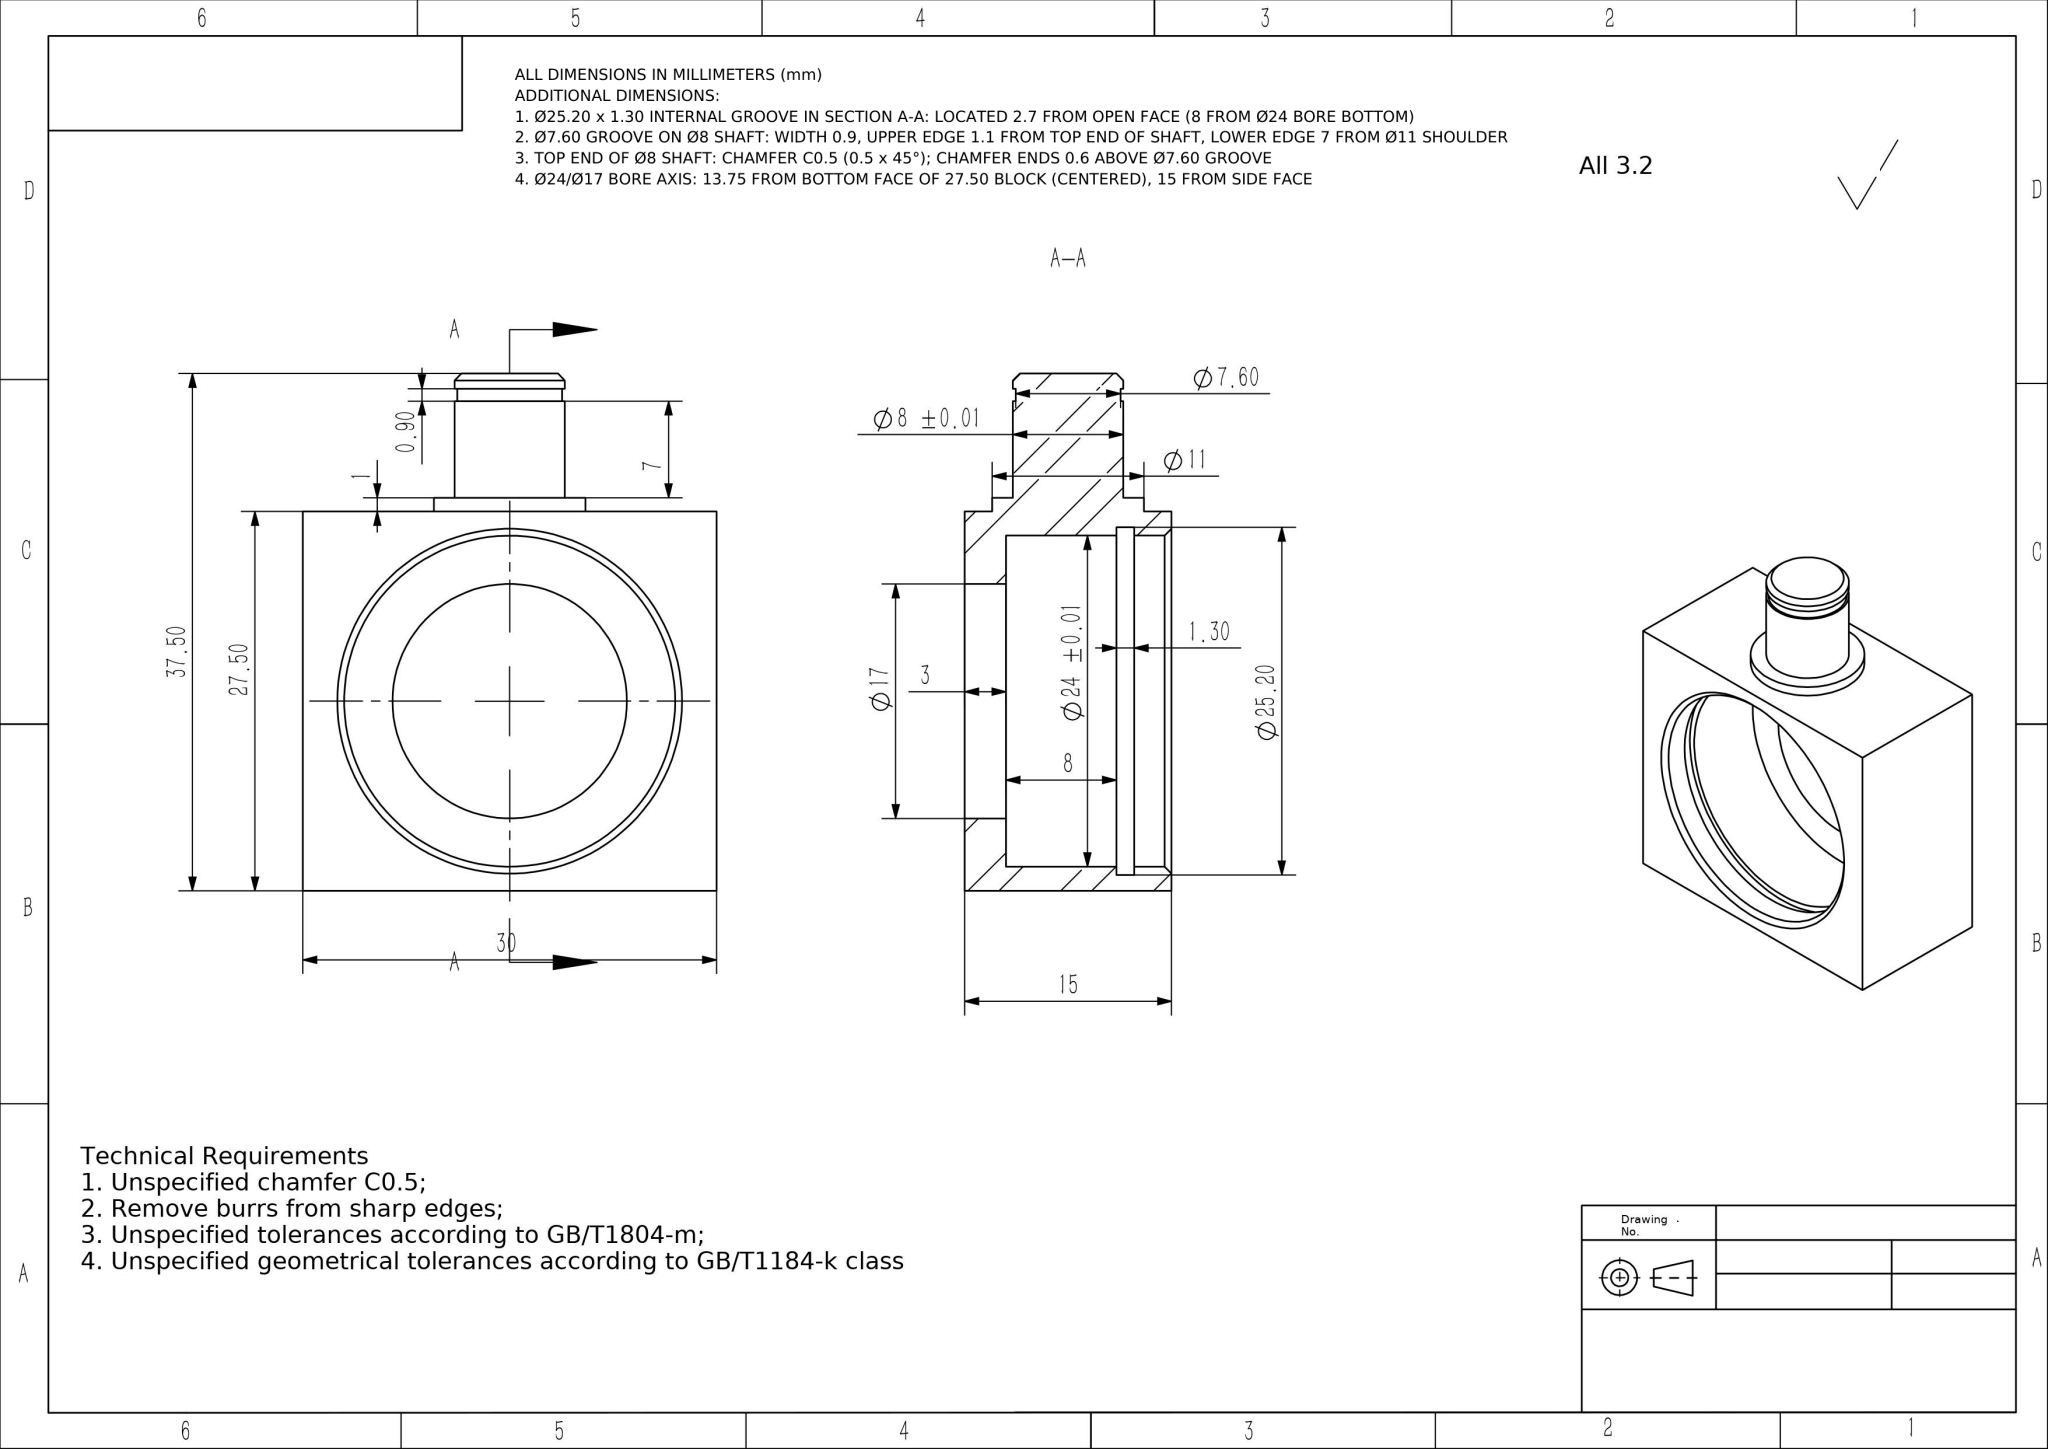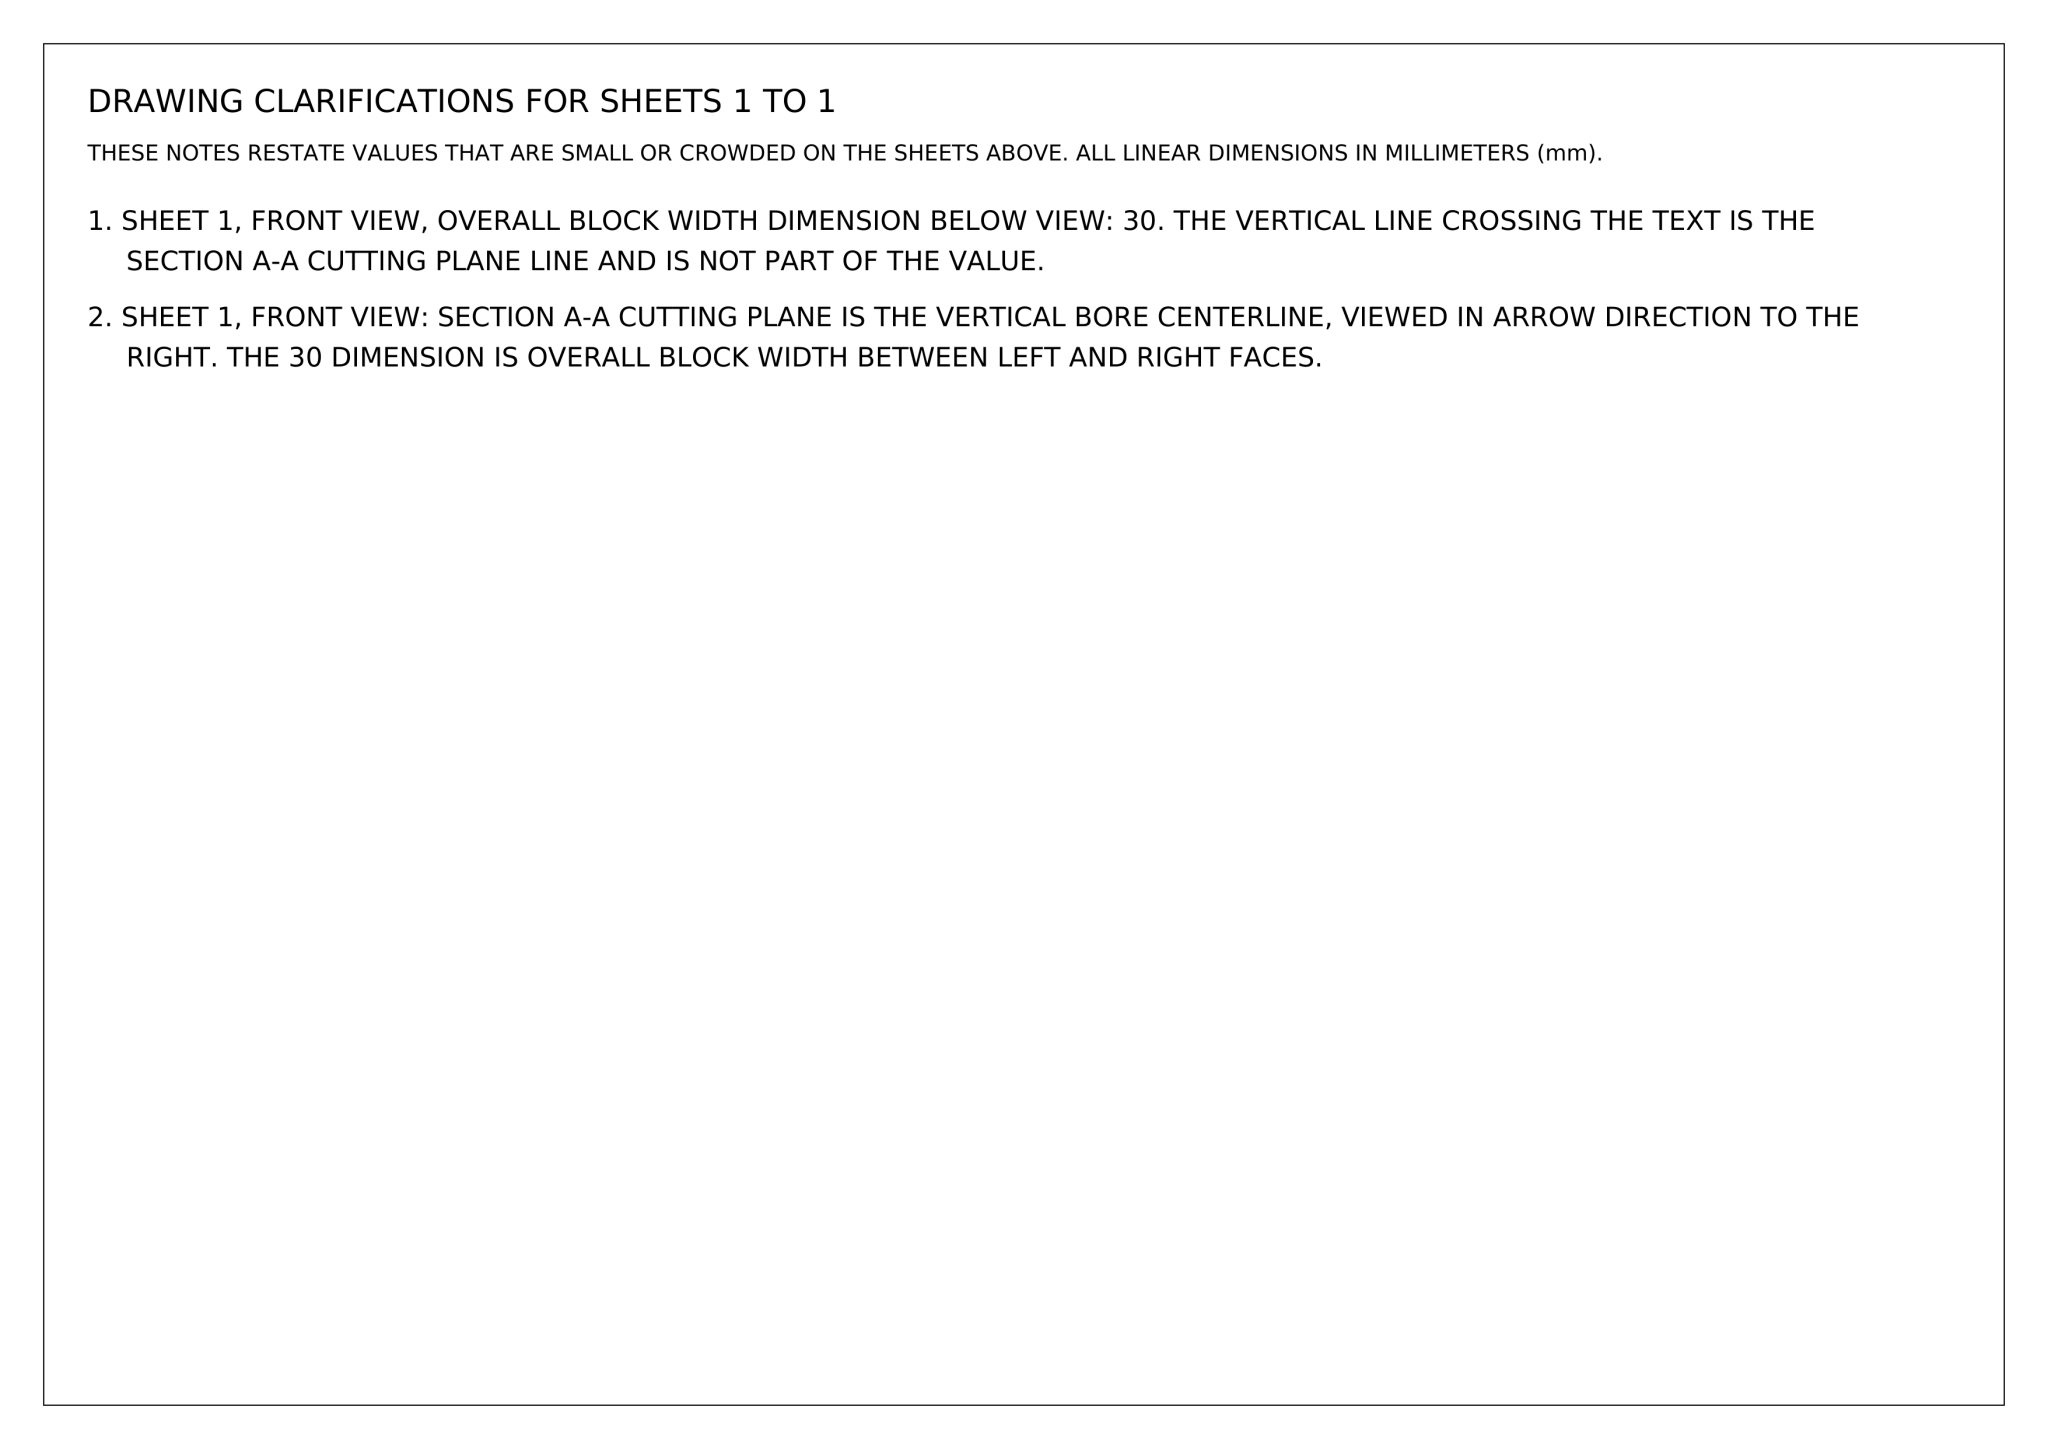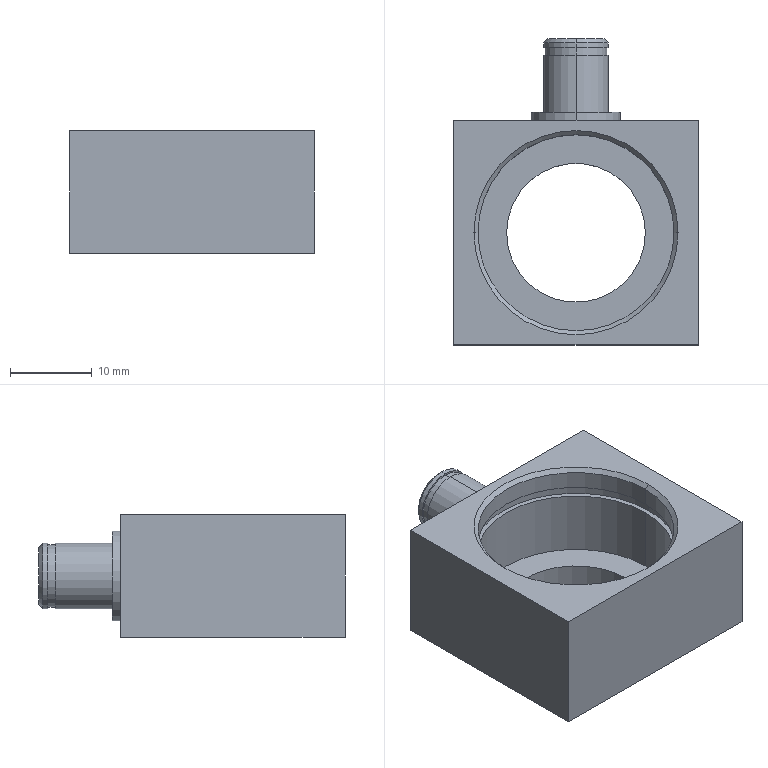Part | NX | mm | 1 solid | 33 faces | box 30 x 37.5 x 15 mm | volume 6736 mm3 | cylinder 16 | plane 13 | cone 4 | commonest cylinder face diameters 24 x4 8 x4 25.2 x2 17 x2 11 x2 7.6 x2